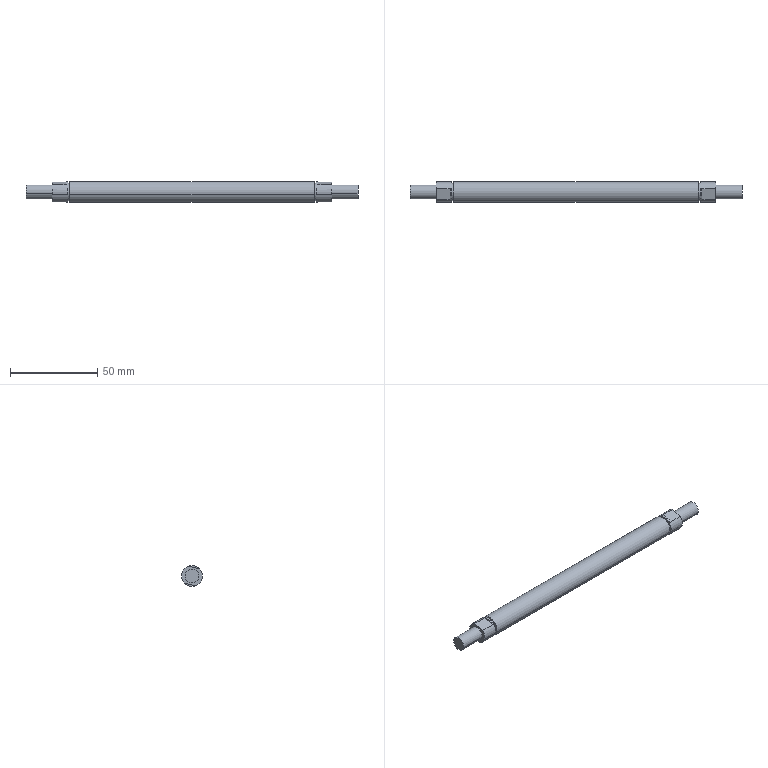Component | SolidWorks | IdlerAssembly4-1_RollerAxis3-1 | 1 solid | 30 faces | box 190 x 12 x 12 mm | volume 19390 mm3 | plane 16 | cylinder 14 | commonest cylinder face diameters 12 x6 10 x4 8 x4
build123d program:
from build123d import *

# Parameters (mm, degrees)
SKETCH1_R           = 6
BOSS_EXTRUDE1_DEPTH = 80
SKETCH3_R           = 4
BOSS_EXTRUDE2_DEPTH = 15
CUT_EXTRUDE7_START  = -8
CUT_EXTRUDE7_DEPTH  = 8
SKETCH20_W          = 1
SKETCH20_H          = 1


with BuildPart() as part:
    # Sketch1 → Boss-Extrude1 (new body)
    with BuildSketch(Plane(origin=(0, 0, 0), x_dir=(1, 0, 0), z_dir=(0, 1, 0))):
        with Locations(Location((0, 0, 0), (0, 0, 270))):
            Circle(SKETCH1_R)
    extrude(amount=BOSS_EXTRUDE1_DEPTH)

    # Sketch3 → Boss-Extrude2 (add)
    with BuildSketch(Plane(origin=(0, 80, 0), x_dir=(1, 0, 0), z_dir=(0, 1, 0))):
        with Locations(Location((0, 0, 0), (0, 0, 270))):
            Circle(SKETCH3_R)
    extrude(amount=BOSS_EXTRUDE2_DEPTH)

    # Sketch17 → Cut-Extrude7 (cut)
    with BuildSketch(Plane(origin=(0, 80, 0), x_dir=(1, 0, 0), z_dir=(0, 1, 0)).offset(CUT_EXTRUDE7_START)):
        with BuildLine():
            Line((-5, 3.317), (-5, -3.317))
            ThreePointArc((-5, -3.317), (-6, 0), (-5, 3.317))
        make_face()
        with BuildLine():
            Line((5, 3.317), (5, -3.317))
            ThreePointArc((5, -3.317), (6, 0), (5, 3.317))
        make_face()
    extrude(amount=CUT_EXTRUDE7_DEPTH, mode=Mode.SUBTRACT)

    # Sketch20 → Cut-Revolve1 (revolve, cut)
    with BuildSketch(Plane(origin=(0, 0, 0), x_dir=(0, 0, -1), z_dir=(1, 0, 0)), mode=Mode.PRIVATE) as cut_revolve1_sk:
        with Locations((5.5, 70.5)):
            Rectangle(SKETCH20_W, SKETCH20_H)
    revolve(cut_revolve1_sk.sketch.rotate(Axis((0, 95, 0), (0, -1, 0)), 180), axis=Axis((0, 95, 0), (0, -1, 0)), mode=Mode.SUBTRACT)

    # Mirror1: part across plane


with BuildPart() as part_1:
    add(part.part)
    add(part.part.mirror(Plane.ZX))


solid = part_1.part

# Placed as in the assembly
solid = solid.moved(Location((-244.97, -95, 30), (-75.719, 0, -90)))
STEP:
#1=COLOUR_RGB('',0.7922,0.8196,0.9333);
#2=FILL_AREA_STYLE_COLOUR('',#1);
#3=FILL_AREA_STYLE('',(#2));
#4=SURFACE_STYLE_FILL_AREA(#3);
#5=SURFACE_SIDE_STYLE('',(#4));
#6=SURFACE_STYLE_USAGE(.BOTH.,#5);
#7=PRESENTATION_STYLE_ASSIGNMENT((#6));
#8=CARTESIAN_POINT('',(-12.4,-3.931,1.133));
#9=VERTEX_POINT('',#8);
#10=CARTESIAN_POINT('',(-12.4,-3.549,1.23));
#11=VERTEX_POINT('',#10);
#12=CARTESIAN_POINT('',(-12.4,-3.74,1.181));
#13=DIRECTION('',(1.,0.,0.));
#14=DIRECTION('',(0.,0.9691,0.2467));
#15=AXIS2_PLACEMENT_3D('',#12,#13,#14);
#16=CIRCLE('',#15,0.1969);
#17=EDGE_CURVE('',#9,#11,#16,.T.);
#18=ORIENTED_EDGE('',*,*,#17,.F.);
#19=CARTESIAN_POINT('',(-12.44,-3.931,1.133));
#20=VERTEX_POINT('',#19);
#21=CARTESIAN_POINT('',(-13.385,-3.931,1.133));
#22=DIRECTION('',(-1.,-0.,-0.));
#23=VECTOR('',#22,39.37);
#24=LINE('',#21,#23);
#25=EDGE_CURVE('',#9,#20,#24,.T.);
#26=ORIENTED_EDGE('',*,*,#25,.T.);
#27=CARTESIAN_POINT('',(-12.44,-3.549,1.23));
#28=VERTEX_POINT('',#27);
#29=CARTESIAN_POINT('',(-12.44,-3.74,1.181));
#30=DIRECTION('',(1.,0.,0.));
#31=DIRECTION('',(0.,0.9691,0.2467));
#32=AXIS2_PLACEMENT_3D('',#29,#30,#31);
#33=CIRCLE('',#32,0.1969);
#34=EDGE_CURVE('',#20,#28,#33,.T.);
#35=ORIENTED_EDGE('',*,*,#34,.T.);
#36=CARTESIAN_POINT('',(-13.385,-3.549,1.23));
#37=DIRECTION('',(-1.,-0.,-0.));
#38=VECTOR('',#37,39.37);
#39=LINE('',#36,#38);
#40=EDGE_CURVE('',#11,#28,#39,.T.);
#41=ORIENTED_EDGE('',*,*,#40,.F.);
#42=EDGE_LOOP('',(#18,#26,#35,#41));
#43=FACE_OUTER_BOUND('',#42,.T.);
#44=CARTESIAN_POINT('',(-13.385,-3.74,1.181));
#45=DIRECTION('',(-1.,-0.,-0.));
#46=DIRECTION('',(0.,0.9691,0.2467));
#47=AXIS2_PLACEMENT_3D('',#44,#45,#46);
#48=CYLINDRICAL_SURFACE('',#47,0.1969);
#49=ADVANCED_FACE('',(#43),#48,.T.);
#50=CARTESIAN_POINT('',(-13.385,-3.893,1.142));
#51=VERTEX_POINT('',#50);
#52=CARTESIAN_POINT('',(-13.385,-3.588,1.22));
#53=VERTEX_POINT('',#52);
#54=CARTESIAN_POINT('',(-13.385,-3.74,1.181));
#55=DIRECTION('',(1.,0.,0.));
#56=DIRECTION('',(0.,0.9691,0.2467));
#57=AXIS2_PLACEMENT_3D('',#54,#55,#56);
#58=CIRCLE('',#57,0.1575);
#59=EDGE_CURVE('',#51,#53,#58,.T.);
#60=ORIENTED_EDGE('',*,*,#59,.T.);
#61=CARTESIAN_POINT('',(-12.794,-3.588,1.22));
#62=VERTEX_POINT('',#61);
#63=CARTESIAN_POINT('',(-13.385,-3.588,1.22));
#64=DIRECTION('',(1.,0.,0.));
#65=VECTOR('',#64,39.37);
#66=LINE('',#63,#65);
#67=EDGE_CURVE('',#53,#62,#66,.T.);
#68=ORIENTED_EDGE('',*,*,#67,.T.);
#69=CARTESIAN_POINT('',(-12.794,-3.893,1.142));
#70=VERTEX_POINT('',#69);
#71=CARTESIAN_POINT('',(-12.794,-3.74,1.181));
#72=DIRECTION('',(1.,0.,0.));
#73=DIRECTION('',(0.,0.9691,0.2467));
#74=AXIS2_PLACEMENT_3D('',#71,#72,#73);
#75=CIRCLE('',#74,0.1575);
#76=EDGE_CURVE('',#70,#62,#75,.T.);
#77=ORIENTED_EDGE('',*,*,#76,.F.);
#78=CARTESIAN_POINT('',(-13.385,-3.893,1.142));
#79=DIRECTION('',(1.,0.,0.));
#80=VECTOR('',#79,39.37);
#81=LINE('',#78,#80);
#82=EDGE_CURVE('',#51,#70,#81,.T.);
#83=ORIENTED_EDGE('',*,*,#82,.F.);
#84=EDGE_LOOP('',(#60,#68,#77,#83));
#85=FACE_OUTER_BOUND('',#84,.T.);
#86=CARTESIAN_POINT('',(-13.385,-3.74,1.181));
#87=DIRECTION('',(1.,0.,0.));
#88=DIRECTION('',(0.,-0.9691,-0.2467));
#89=AXIS2_PLACEMENT_3D('',#86,#87,#88);
#90=CYLINDRICAL_SURFACE('',#89,0.1575);
#91=ADVANCED_FACE('',(#85),#90,.T.);
#92=CARTESIAN_POINT('',(-12.794,-3.565,1.023));
#93=VERTEX_POINT('',#92);
#94=CARTESIAN_POINT('',(-12.794,-3.511,1.239));
#95=VERTEX_POINT('',#94);
#96=CARTESIAN_POINT('',(-12.794,-3.74,1.181));
#97=DIRECTION('',(1.,0.,0.));
#98=DIRECTION('',(0.,0.9691,0.2467));
#99=AXIS2_PLACEMENT_3D('',#96,#97,#98);
#100=CIRCLE('',#99,0.2362);
#101=EDGE_CURVE('',#93,#95,#100,.T.);
#102=ORIENTED_EDGE('',*,*,#101,.T.);
#103=CARTESIAN_POINT('',(-12.44,-3.511,1.239));
#104=VERTEX_POINT('',#103);
#105=CARTESIAN_POINT('',(-12.794,-3.511,1.239));
#106=DIRECTION('',(1.,0.,0.));
#107=VECTOR('',#106,39.37);
#108=LINE('',#105,#107);
#109=EDGE_CURVE('',#95,#104,#108,.T.);
#110=ORIENTED_EDGE('',*,*,#109,.T.);
#111=CARTESIAN_POINT('',(-12.44,-3.969,1.123));
#112=VERTEX_POINT('',#111);
#113=CARTESIAN_POINT('',(-12.44,-3.74,1.181));
#114=DIRECTION('',(1.,0.,0.));
#115=DIRECTION('',(0.,0.9691,0.2467));
#116=AXIS2_PLACEMENT_3D('',#113,#114,#115);
#117=CIRCLE('',#116,0.2362);
#118=EDGE_CURVE('',#112,#104,#117,.T.);
#119=ORIENTED_EDGE('',*,*,#118,.F.);
#120=CARTESIAN_POINT('',(-12.794,-3.969,1.123));
#121=VERTEX_POINT('',#120);
#122=CARTESIAN_POINT('',(-12.794,-3.969,1.123));
#123=DIRECTION('',(1.,0.,0.));
#124=VECTOR('',#123,39.37);
#125=LINE('',#122,#124);
#126=EDGE_CURVE('',#121,#112,#125,.T.);
#127=ORIENTED_EDGE('',*,*,#126,.F.);
#128=CARTESIAN_POINT('',(-12.794,-3.818,0.9581));
#129=VERTEX_POINT('',#128);
#130=CARTESIAN_POINT('',(-12.794,-3.74,1.181));
#131=DIRECTION('',(1.,0.,0.));
#132=DIRECTION('',(0.,0.9691,0.2467));
#133=AXIS2_PLACEMENT_3D('',#130,#131,#132);
#134=CIRCLE('',#133,0.2362);
#135=EDGE_CURVE('',#121,#129,#134,.T.);
#136=ORIENTED_EDGE('',*,*,#135,.T.);
#137=CARTESIAN_POINT('',(-12.479,-3.818,0.9581));
#138=VERTEX_POINT('',#137);
#139=CARTESIAN_POINT('',(-12.479,-3.818,0.9581));
#140=DIRECTION('',(-1.,-0.,-0.));
#141=VECTOR('',#140,39.37);
#142=LINE('',#139,#141);
#143=EDGE_CURVE('',#138,#129,#142,.T.);
#144=ORIENTED_EDGE('',*,*,#143,.F.);
#145=CARTESIAN_POINT('',(-12.479,-3.565,1.023));
#146=VERTEX_POINT('',#145);
#147=CARTESIAN_POINT('',(-12.479,-3.74,1.181));
#148=DIRECTION('',(1.,0.,0.));
#149=DIRECTION('',(0.,0.9691,0.2467));
#150=AXIS2_PLACEMENT_3D('',#147,#148,#149);
#151=CIRCLE('',#150,0.2362);
#152=EDGE_CURVE('',#138,#146,#151,.T.);
#153=ORIENTED_EDGE('',*,*,#152,.T.);
#154=CARTESIAN_POINT('',(-12.479,-3.565,1.023));
#155=DIRECTION('',(-1.,-0.,-0.));
#156=VECTOR('',#155,39.37);
#157=LINE('',#154,#156);
#158=EDGE_CURVE('',#146,#93,#157,.T.);
#159=ORIENTED_EDGE('',*,*,#158,.T.);
#160=EDGE_LOOP('',(#102,#110,#119,#127,#136,#144,#153,#159));
#161=FACE_OUTER_BOUND('',#160,.T.);
#162=CARTESIAN_POINT('',(-12.794,-3.74,1.181));
#163=DIRECTION('',(1.,0.,0.));
#164=DIRECTION('',(0.,-0.9691,-0.2467));
#165=AXIS2_PLACEMENT_3D('',#162,#163,#164);
#166=CYLINDRICAL_SURFACE('',#165,0.2362);
#167=ADVANCED_FACE('',(#161),#166,.T.);
#168=CARTESIAN_POINT('',(-6.889,-3.511,1.239));
#169=VERTEX_POINT('',#168);
#170=CARTESIAN_POINT('',(-6.889,-3.969,1.123));
#171=VERTEX_POINT('',#170);
#172=CARTESIAN_POINT('',(-6.889,-3.74,1.181));
#173=DIRECTION('',(1.,0.,0.));
#174=DIRECTION('',(0.,0.9691,0.2467));
#175=AXIS2_PLACEMENT_3D('',#172,#173,#174);
#176=CIRCLE('',#175,0.2362);
#177=EDGE_CURVE('',#169,#171,#176,.T.);
#178=ORIENTED_EDGE('',*,*,#177,.F.);
#179=CARTESIAN_POINT('',(-12.4,-3.511,1.239));
#180=VERTEX_POINT('',#179);
#181=CARTESIAN_POINT('',(-6.495,-3.511,1.239));
#182=DIRECTION('',(-1.,-0.,-0.));
#183=VECTOR('',#182,39.37);
#184=LINE('',#181,#183);
#185=EDGE_CURVE('',#169,#180,#184,.T.);
#186=ORIENTED_EDGE('',*,*,#185,.T.);
#187=CARTESIAN_POINT('',(-12.4,-3.969,1.123));
#188=VERTEX_POINT('',#187);
#189=CARTESIAN_POINT('',(-12.4,-3.74,1.181));
#190=DIRECTION('',(1.,0.,0.));
#191=DIRECTION('',(0.,0.9691,0.2467));
#192=AXIS2_PLACEMENT_3D('',#189,#190,#191);
#193=CIRCLE('',#192,0.2362);
#194=EDGE_CURVE('',#180,#188,#193,.T.);
#195=ORIENTED_EDGE('',*,*,#194,.T.);
#196=CARTESIAN_POINT('',(-6.495,-3.969,1.123));
#197=DIRECTION('',(-1.,-0.,-0.));
#198=VECTOR('',#197,39.37);
#199=LINE('',#196,#198);
#200=EDGE_CURVE('',#171,#188,#199,.T.);
#201=ORIENTED_EDGE('',*,*,#200,.F.);
#202=EDGE_LOOP('',(#178,#186,#195,#201));
#203=FACE_OUTER_BOUND('',#202,.T.);
#204=CARTESIAN_POINT('',(-6.495,-3.74,1.181));
#205=DIRECTION('',(-1.,-0.,-0.));
#206=DIRECTION('',(0.,-0.9691,-0.2467));
#207=AXIS2_PLACEMENT_3D('',#204,#205,#206);
#208=CYLINDRICAL_SURFACE('',#207,0.2362);
#209=ADVANCED_FACE('',(#203),#208,.T.);
#210=CARTESIAN_POINT('',(-6.889,-3.549,1.23));
#211=VERTEX_POINT('',#210);
#212=CARTESIAN_POINT('',(-6.889,-3.931,1.133));
#213=VERTEX_POINT('',#212);
#214=CARTESIAN_POINT('',(-6.889,-3.74,1.181));
#215=DIRECTION('',(1.,0.,0.));
#216=DIRECTION('',(0.,0.9691,0.2467));
#217=AXIS2_PLACEMENT_3D('',#214,#215,#216);
#218=CIRCLE('',#217,0.1969);
#219=EDGE_CURVE('',#211,#213,#218,.T.);
#220=ORIENTED_EDGE('',*,*,#219,.T.);
#221=CARTESIAN_POINT('',(-6.849,-3.931,1.133));
#222=VERTEX_POINT('',#221);
#223=CARTESIAN_POINT('',(-5.904,-3.931,1.133));
#224=DIRECTION('',(1.,0.,0.));
#225=VECTOR('',#224,39.37);
#226=LINE('',#223,#225);
#227=EDGE_CURVE('',#213,#222,#226,.T.);
#228=ORIENTED_EDGE('',*,*,#227,.T.);
#229=CARTESIAN_POINT('',(-6.849,-3.549,1.23));
#230=VERTEX_POINT('',#229);
#231=CARTESIAN_POINT('',(-6.849,-3.74,1.181));
#232=DIRECTION('',(1.,0.,0.));
#233=DIRECTION('',(0.,0.9691,0.2467));
#234=AXIS2_PLACEMENT_3D('',#231,#232,#233);
#235=CIRCLE('',#234,0.1969);
#236=EDGE_CURVE('',#230,#222,#235,.T.);
#237=ORIENTED_EDGE('',*,*,#236,.F.);
#238=CARTESIAN_POINT('',(-5.904,-3.549,1.23));
#239=DIRECTION('',(1.,0.,0.));
#240=VECTOR('',#239,39.37);
#241=LINE('',#238,#240);
#242=EDGE_CURVE('',#211,#230,#241,.T.);
#243=ORIENTED_EDGE('',*,*,#242,.F.);
#244=EDGE_LOOP('',(#220,#228,#237,#243));
#245=FACE_OUTER_BOUND('',#244,.T.);
#246=CARTESIAN_POINT('',(-5.904,-3.74,1.181));
#247=DIRECTION('',(1.,0.,0.));
#248=DIRECTION('',(0.,0.9691,0.2467));
#249=AXIS2_PLACEMENT_3D('',#246,#247,#248);
#250=CYLINDRICAL_SURFACE('',#249,0.1969);
#251=ADVANCED_FACE('',(#245),#250,.T.);
#252=CARTESIAN_POINT('',(-5.904,-3.588,1.22));
#253=VERTEX_POINT('',#252);
#254=CARTESIAN_POINT('',(-5.904,-3.893,1.142));
#255=VERTEX_POINT('',#254);
#256=CARTESIAN_POINT('',(-5.904,-3.74,1.181));
#257=DIRECTION('',(1.,0.,0.));
#258=DIRECTION('',(0.,0.9691,0.2467));
#259=AXIS2_PLACEMENT_3D('',#256,#257,#258);
#260=CIRCLE('',#259,0.1575);
#261=EDGE_CURVE('',#253,#255,#260,.T.);
#262=ORIENTED_EDGE('',*,*,#261,.F.);
#263=CARTESIAN_POINT('',(-6.495,-3.588,1.22));
#264=VERTEX_POINT('',#263);
#265=CARTESIAN_POINT('',(-5.904,-3.588,1.22));
#266=DIRECTION('',(-1.,-0.,-0.));
#267=VECTOR('',#266,39.37);
#268=LINE('',#265,#267);
#269=EDGE_CURVE('',#253,#264,#268,.T.);
#270=ORIENTED_EDGE('',*,*,#269,.T.);
#271=CARTESIAN_POINT('',(-6.495,-3.893,1.142));
#272=VERTEX_POINT('',#271);
#273=CARTESIAN_POINT('',(-6.495,-3.74,1.181));
#274=DIRECTION('',(1.,0.,0.));
#275=DIRECTION('',(0.,0.9691,0.2467));
#276=AXIS2_PLACEMENT_3D('',#273,#274,#275);
#277=CIRCLE('',#276,0.1575);
#278=EDGE_CURVE('',#264,#272,#277,.T.);
#279=ORIENTED_EDGE('',*,*,#278,.T.);
#280=CARTESIAN_POINT('',(-5.904,-3.893,1.142));
#281=DIRECTION('',(-1.,-0.,-0.));
#282=VECTOR('',#281,39.37);
#283=LINE('',#280,#282);
#284=EDGE_CURVE('',#255,#272,#283,.T.);
#285=ORIENTED_EDGE('',*,*,#284,.F.);
#286=EDGE_LOOP('',(#262,#270,#279,#285));
#287=FACE_OUTER_BOUND('',#286,.T.);
#288=CARTESIAN_POINT('',(-5.904,-3.74,1.181));
#289=DIRECTION('',(-1.,-0.,-0.));
#290=DIRECTION('',(0.,-0.9691,-0.2467));
#291=AXIS2_PLACEMENT_3D('',#288,#289,#290);
#292=CYLINDRICAL_SURFACE('',#291,0.1575);
#293=ADVANCED_FACE('',(#287),#292,.T.);
#294=CARTESIAN_POINT('',(-6.495,-3.511,1.239));
#295=VERTEX_POINT('',#294);
#296=CARTESIAN_POINT('',(-6.495,-3.662,1.404));
#297=VERTEX_POINT('',#296);
#298=CARTESIAN_POINT('',(-6.495,-3.74,1.181));
#299=DIRECTION('',(1.,0.,0.));
#300=DIRECTION('',(0.,0.9691,0.2467));
#301=AXIS2_PLACEMENT_3D('',#298,#299,#300);
#302=CIRCLE('',#301,0.2362);
#303=EDGE_CURVE('',#295,#297,#302,.T.);
#304=ORIENTED_EDGE('',*,*,#303,.F.);
#305=CARTESIAN_POINT('',(-6.849,-3.511,1.239));
#306=VERTEX_POINT('',#305);
#307=CARTESIAN_POINT('',(-6.495,-3.511,1.239));
#308=DIRECTION('',(-1.,-0.,-0.));
#309=VECTOR('',#308,39.37);
#310=LINE('',#307,#309);
#311=EDGE_CURVE('',#295,#306,#310,.T.);
#312=ORIENTED_EDGE('',*,*,#311,.T.);
#313=CARTESIAN_POINT('',(-6.849,-3.969,1.123));
#314=VERTEX_POINT('',#313);
#315=CARTESIAN_POINT('',(-6.849,-3.74,1.181));
#316=DIRECTION('',(1.,0.,0.));
#317=DIRECTION('',(0.,0.9691,0.2467));
#318=AXIS2_PLACEMENT_3D('',#315,#316,#317);
#319=CIRCLE('',#318,0.2362);
#320=EDGE_CURVE('',#306,#314,#319,.T.);
#321=ORIENTED_EDGE('',*,*,#320,.T.);
#322=CARTESIAN_POINT('',(-6.495,-3.969,1.123));
#323=VERTEX_POINT('',#322);
#324=CARTESIAN_POINT('',(-6.495,-3.969,1.123));
#325=DIRECTION('',(-1.,-0.,-0.));
#326=VECTOR('',#325,39.37);
#327=LINE('',#324,#326);
#328=EDGE_CURVE('',#323,#314,#327,.T.);
#329=ORIENTED_EDGE('',*,*,#328,.F.);
#330=CARTESIAN_POINT('',(-6.495,-3.915,1.34));
#331=VERTEX_POINT('',#330);
#332=CARTESIAN_POINT('',(-6.495,-3.74,1.181));
#333=DIRECTION('',(1.,0.,0.));
#334=DIRECTION('',(0.,0.9691,0.2467));
#335=AXIS2_PLACEMENT_3D('',#332,#333,#334);
#336=CIRCLE('',#335,0.2362);
#337=EDGE_CURVE('',#331,#323,#336,.T.);
#338=ORIENTED_EDGE('',*,*,#337,.F.);
#339=CARTESIAN_POINT('',(-6.81,-3.915,1.34));
#340=VERTEX_POINT('',#339);
#341=CARTESIAN_POINT('',(-6.81,-3.915,1.34));
#342=DIRECTION('',(1.,0.,0.));
#343=VECTOR('',#342,39.37);
#344=LINE('',#341,#343);
#345=EDGE_CURVE('',#340,#331,#344,.T.);
#346=ORIENTED_EDGE('',*,*,#345,.F.);
#347=CARTESIAN_POINT('',(-6.81,-3.662,1.404));
#348=VERTEX_POINT('',#347);
#349=CARTESIAN_POINT('',(-6.81,-3.74,1.181));
#350=DIRECTION('',(1.,0.,0.));
#351=DIRECTION('',(0.,0.9691,0.2467));
#352=AXIS2_PLACEMENT_3D('',#349,#350,#351);
#353=CIRCLE('',#352,0.2362);
#354=EDGE_CURVE('',#348,#340,#353,.T.);
#355=ORIENTED_EDGE('',*,*,#354,.F.);
#356=CARTESIAN_POINT('',(-6.81,-3.662,1.404));
#357=DIRECTION('',(1.,0.,0.));
#358=VECTOR('',#357,39.37);
#359=LINE('',#356,#358);
#360=EDGE_CURVE('',#348,#297,#359,.T.);
#361=ORIENTED_EDGE('',*,*,#360,.T.);
#362=EDGE_LOOP('',(#304,#312,#321,#329,#338,#346,#355,#361));
#363=FACE_OUTER_BOUND('',#362,.T.);
#364=CARTESIAN_POINT('',(-6.495,-3.74,1.181));
#365=DIRECTION('',(-1.,-0.,-0.));
#366=DIRECTION('',(0.,-0.9691,-0.2467));
#367=AXIS2_PLACEMENT_3D('',#364,#365,#366);
#368=CYLINDRICAL_SURFACE('',#367,0.2362);
#369=ADVANCED_FACE('',(#363),#368,.T.);
#370=ORIENTED_EDGE('',*,*,#311,.F.);
#371=CARTESIAN_POINT('',(-6.495,-3.565,1.023));
#372=VERTEX_POINT('',#371);
#373=CARTESIAN_POINT('',(-6.495,-3.74,1.181));
#374=DIRECTION('',(1.,0.,0.));
#375=DIRECTION('',(0.,0.9691,0.2467));
#376=AXIS2_PLACEMENT_3D('',#373,#374,#375);
#377=CIRCLE('',#376,0.2362);
#378=EDGE_CURVE('',#372,#295,#377,.T.);
#379=ORIENTED_EDGE('',*,*,#378,.F.);
#380=CARTESIAN_POINT('',(-6.81,-3.565,1.023));
#381=VERTEX_POINT('',#380);
#382=CARTESIAN_POINT('',(-6.81,-3.565,1.023));
#383=DIRECTION('',(1.,0.,0.));
#384=VECTOR('',#383,39.37);
#385=LINE('',#382,#384);
#386=EDGE_CURVE('',#381,#372,#385,.T.);
#387=ORIENTED_EDGE('',*,*,#386,.F.);
#388=CARTESIAN_POINT('',(-6.81,-3.818,0.9581));
#389=VERTEX_POINT('',#388);
#390=CARTESIAN_POINT('',(-6.81,-3.74,1.181));
#391=DIRECTION('',(1.,0.,0.));
#392=DIRECTION('',(0.,0.9691,0.2467));
#393=AXIS2_PLACEMENT_3D('',#390,#391,#392);
#394=CIRCLE('',#393,0.2362);
#395=EDGE_CURVE('',#389,#381,#394,.T.);
#396=ORIENTED_EDGE('',*,*,#395,.F.);
#397=CARTESIAN_POINT('',(-6.495,-3.818,0.9581));
#398=VERTEX_POINT('',#397);
#399=CARTESIAN_POINT('',(-6.81,-3.818,0.9581));
#400=DIRECTION('',(1.,0.,0.));
#401=VECTOR('',#400,39.37);
#402=LINE('',#399,#401);
#403=EDGE_CURVE('',#389,#398,#402,.T.);
#404=ORIENTED_EDGE('',*,*,#403,.T.);
#405=CARTESIAN_POINT('',(-6.495,-3.74,1.181));
#406=DIRECTION('',(1.,0.,0.));
#407=DIRECTION('',(0.,0.9691,0.2467));
#408=AXIS2_PLACEMENT_3D('',#405,#406,#407);
#409=CIRCLE('',#408,0.2362);
#410=EDGE_CURVE('',#323,#398,#409,.T.);
#411=ORIENTED_EDGE('',*,*,#410,.F.);
#412=ORIENTED_EDGE('',*,*,#328,.T.);
#413=CARTESIAN_POINT('',(-6.849,-3.74,1.181));
#414=DIRECTION('',(1.,0.,0.));
#415=DIRECTION('',(0.,0.9691,0.2467));
#416=AXIS2_PLACEMENT_3D('',#413,#414,#415);
#417=CIRCLE('',#416,0.2362);
#418=EDGE_CURVE('',#314,#306,#417,.T.);
#419=ORIENTED_EDGE('',*,*,#418,.T.);
#420=EDGE_LOOP('',(#370,#379,#387,#396,#404,#411,#412,#419));
#421=FACE_OUTER_BOUND('',#420,.T.);
#422=CARTESIAN_POINT('',(-6.495,-3.74,1.181));
#423=DIRECTION('',(-1.,-0.,-0.));
#424=DIRECTION('',(0.,-0.9691,-0.2467));
#425=AXIS2_PLACEMENT_3D('',#422,#423,#424);
#426=CYLINDRICAL_SURFACE('',#425,0.2362);
#427=ADVANCED_FACE('',(#421),#426,.T.);
#428=CARTESIAN_POINT('',(-6.495,-3.818,0.9581));
#429=DIRECTION('',(0.,-0.9691,-0.2467));
#430=VECTOR('',#429,39.37);
#431=LINE('',#428,#430);
#432=EDGE_CURVE('',#372,#398,#431,.T.);
#433=ORIENTED_EDGE('',*,*,#432,.F.);
#434=ORIENTED_EDGE('',*,*,#378,.T.);
#435=ORIENTED_EDGE('',*,*,#303,.T.);
#436=CARTESIAN_POINT('',(-6.495,-3.915,1.34));
#437=DIRECTION('',(-0.,0.9691,0.2467));
#438=VECTOR('',#437,39.37);
#439=LINE('',#436,#438);
#440=EDGE_CURVE('',#331,#297,#439,.T.);
#441=ORIENTED_EDGE('',*,*,#440,.F.);
#442=ORIENTED_EDGE('',*,*,#337,.T.);
#443=ORIENTED_EDGE('',*,*,#410,.T.);
#444=EDGE_LOOP('',(#433,#434,#435,#441,#442,#443));
#445=FACE_OUTER_BOUND('',#444,.T.);
#446=CARTESIAN_POINT('',(-6.495,-3.74,1.181));
#447=DIRECTION('',(1.,0.,0.));
#448=DIRECTION('',(0.,0.9691,0.2467));
#449=AXIS2_PLACEMENT_3D('',#446,#447,#448);
#450=CIRCLE('',#449,0.1575);
#451=EDGE_CURVE('',#272,#264,#450,.T.);
#452=ORIENTED_EDGE('',*,*,#451,.F.);
#453=ORIENTED_EDGE('',*,*,#278,.F.);
#454=EDGE_LOOP('',(#452,#453));
#455=FACE_BOUND('',#454,.T.);
#456=CARTESIAN_POINT('',(-6.495,-3.74,1.181));
#457=DIRECTION('',(1.,0.,0.));
#458=DIRECTION('',(-0.,0.9691,0.2467));
#459=AXIS2_PLACEMENT_3D('',#456,#457,#458);
#460=PLANE('',#459);
#461=ADVANCED_FACE('',(#445,#455),#460,.T.);
#462=ORIENTED_EDGE('',*,*,#269,.F.);
#463=CARTESIAN_POINT('',(-5.904,-3.74,1.181));
#464=DIRECTION('',(1.,0.,0.));
#465=DIRECTION('',(0.,0.9691,0.2467));
#466=AXIS2_PLACEMENT_3D('',#463,#464,#465);
#467=CIRCLE('',#466,0.1575);
#468=EDGE_CURVE('',#255,#253,#467,.T.);
#469=ORIENTED_EDGE('',*,*,#468,.F.);
#470=ORIENTED_EDGE('',*,*,#284,.T.);
#471=ORIENTED_EDGE('',*,*,#451,.T.);
#472=EDGE_LOOP('',(#462,#469,#470,#471));
#473=FACE_OUTER_BOUND('',#472,.T.);
#474=CARTESIAN_POINT('',(-5.904,-3.74,1.181));
#475=DIRECTION('',(-1.,-0.,-0.));
#476=DIRECTION('',(0.,-0.9691,-0.2467));
#477=AXIS2_PLACEMENT_3D('',#474,#475,#476);
#478=CYLINDRICAL_SURFACE('',#477,0.1575);
#479=ADVANCED_FACE('',(#473),#478,.T.);
#480=ORIENTED_EDGE('',*,*,#468,.T.);
#481=ORIENTED_EDGE('',*,*,#261,.T.);
#482=EDGE_LOOP('',(#480,#481));
#483=FACE_OUTER_BOUND('',#482,.T.);
#484=CARTESIAN_POINT('',(-5.904,-3.74,1.181));
#485=DIRECTION('',(1.,0.,0.));
#486=DIRECTION('',(-0.,0.9691,0.2467));
#487=AXIS2_PLACEMENT_3D('',#484,#485,#486);
#488=PLANE('',#487);
#489=ADVANCED_FACE('',(#483),#488,.T.);
#490=ORIENTED_EDGE('',*,*,#440,.T.);
#491=ORIENTED_EDGE('',*,*,#360,.F.);
#492=CARTESIAN_POINT('',(-6.81,-3.915,1.34));
#493=DIRECTION('',(-0.,0.9691,0.2467));
#494=VECTOR('',#493,39.37);
#495=LINE('',#492,#494);
#496=EDGE_CURVE('',#340,#348,#495,.T.);
#497=ORIENTED_EDGE('',*,*,#496,.F.);
#498=ORIENTED_EDGE('',*,*,#345,.T.);
#499=EDGE_LOOP('',(#490,#491,#497,#498));
#500=FACE_OUTER_BOUND('',#499,.T.);
#501=CARTESIAN_POINT('',(-6.81,-3.915,1.34));
#502=DIRECTION('',(0.,0.2467,-0.9691));
#503=DIRECTION('',(-0.,0.9691,0.2467));
#504=AXIS2_PLACEMENT_3D('',#501,#502,#503);
#505=PLANE('',#504);
#506=ADVANCED_FACE('',(#500),#505,.F.);
#507=ORIENTED_EDGE('',*,*,#354,.T.);
#508=ORIENTED_EDGE('',*,*,#496,.T.);
#509=EDGE_LOOP('',(#507,#508));
#510=FACE_OUTER_BOUND('',#509,.T.);
#511=CARTESIAN_POINT('',(-6.81,-3.74,1.181));
#512=DIRECTION('',(1.,0.,0.));
#513=DIRECTION('',(-0.,0.9691,0.2467));
#514=AXIS2_PLACEMENT_3D('',#511,#512,#513);
#515=PLANE('',#514);
#516=ADVANCED_FACE('',(#510),#515,.T.);
#517=ORIENTED_EDGE('',*,*,#432,.T.);
#518=ORIENTED_EDGE('',*,*,#403,.F.);
#519=CARTESIAN_POINT('',(-6.81,-3.818,0.9581));
#520=DIRECTION('',(0.,-0.9691,-0.2467));
#521=VECTOR('',#520,39.37);
#522=LINE('',#519,#521);
#523=EDGE_CURVE('',#381,#389,#522,.T.);
#524=ORIENTED_EDGE('',*,*,#523,.F.);
#525=ORIENTED_EDGE('',*,*,#386,.T.);
#526=EDGE_LOOP('',(#517,#518,#524,#525));
#527=FACE_OUTER_BOUND('',#526,.T.);
#528=CARTESIAN_POINT('',(-6.81,-3.818,0.9581));
#529=DIRECTION('',(-0.,-0.2467,0.9691));
#530=DIRECTION('',(0.,-0.9691,-0.2467));
#531=AXIS2_PLACEMENT_3D('',#528,#529,#530);
#532=PLANE('',#531);
#533=ADVANCED_FACE('',(#527),#532,.F.);
#534=ORIENTED_EDGE('',*,*,#395,.T.);
#535=ORIENTED_EDGE('',*,*,#523,.T.);
#536=EDGE_LOOP('',(#534,#535));
#537=FACE_OUTER_BOUND('',#536,.T.);
#538=CARTESIAN_POINT('',(-6.81,-3.74,1.181));
#539=DIRECTION('',(1.,0.,0.));
#540=DIRECTION('',(-0.,0.9691,0.2467));
#541=AXIS2_PLACEMENT_3D('',#538,#539,#540);
#542=PLANE('',#541);
#543=ADVANCED_FACE('',(#537),#542,.T.);
#544=CARTESIAN_POINT('',(-6.889,-3.74,1.181));
#545=DIRECTION('',(1.,0.,0.));
#546=DIRECTION('',(0.,0.9691,0.2467));
#547=AXIS2_PLACEMENT_3D('',#544,#545,#546);
#548=CIRCLE('',#547,0.2362);
#549=EDGE_CURVE('',#171,#169,#548,.T.);
#550=ORIENTED_EDGE('',*,*,#549,.T.);
#551=ORIENTED_EDGE('',*,*,#177,.T.);
#552=EDGE_LOOP('',(#550,#551));
#553=FACE_OUTER_BOUND('',#552,.T.);
#554=ORIENTED_EDGE('',*,*,#219,.F.);
#555=CARTESIAN_POINT('',(-6.889,-3.74,1.181));
#556=DIRECTION('',(1.,0.,0.));
#557=DIRECTION('',(0.,0.9691,0.2467));
#558=AXIS2_PLACEMENT_3D('',#555,#556,#557);
#559=CIRCLE('',#558,0.1969);
#560=EDGE_CURVE('',#213,#211,#559,.T.);
#561=ORIENTED_EDGE('',*,*,#560,.F.);
#562=EDGE_LOOP('',(#554,#561));
#563=FACE_BOUND('',#562,.T.);
#564=CARTESIAN_POINT('',(-6.889,-3.969,1.123));
#565=DIRECTION('',(1.,0.,0.));
#566=DIRECTION('',(-0.,0.9691,0.2467));
#567=AXIS2_PLACEMENT_3D('',#564,#565,#566);
#568=PLANE('',#567);
#569=ADVANCED_FACE('',(#553,#563),#568,.T.);
#570=ORIENTED_EDGE('',*,*,#227,.F.);
#571=ORIENTED_EDGE('',*,*,#560,.T.);
#572=ORIENTED_EDGE('',*,*,#242,.T.);
#573=CARTESIAN_POINT('',(-6.849,-3.74,1.181));
#574=DIRECTION('',(1.,0.,0.));
#575=DIRECTION('',(0.,0.9691,0.2467));
#576=AXIS2_PLACEMENT_3D('',#573,#574,#575);
#577=CIRCLE('',#576,0.1969);
#578=EDGE_CURVE('',#222,#230,#577,.T.);
#579=ORIENTED_EDGE('',*,*,#578,.F.);
#580=EDGE_LOOP('',(#570,#571,#572,#579));
#581=FACE_OUTER_BOUND('',#580,.T.);
#582=CARTESIAN_POINT('',(-5.904,-3.74,1.181));
#583=DIRECTION('',(1.,0.,0.));
#584=DIRECTION('',(0.,0.9691,0.2467));
#585=AXIS2_PLACEMENT_3D('',#582,#583,#584);
#586=CYLINDRICAL_SURFACE('',#585,0.1969);
#587=ADVANCED_FACE('',(#581),#586,.T.);
#588=ORIENTED_EDGE('',*,*,#236,.T.);
#589=ORIENTED_EDGE('',*,*,#578,.T.);
#590=EDGE_LOOP('',(#588,#589));
#591=FACE_BOUND('',#590,.T.);
#592=ORIENTED_EDGE('',*,*,#418,.F.);
#593=ORIENTED_EDGE('',*,*,#320,.F.);
#594=EDGE_LOOP('',(#592,#593));
#595=FACE_OUTER_BOUND('',#594,.T.);
#596=CARTESIAN_POINT('',(-6.849,-3.969,1.123));
#597=DIRECTION('',(-1.,-0.,-0.));
#598=DIRECTION('',(0.,-0.9691,-0.2467));
#599=AXIS2_PLACEMENT_3D('',#596,#597,#598);
#600=PLANE('',#599);
#601=ADVANCED_FACE('',(#591,#595),#600,.T.);
#602=ORIENTED_EDGE('',*,*,#185,.F.);
#603=ORIENTED_EDGE('',*,*,#549,.F.);
#604=ORIENTED_EDGE('',*,*,#200,.T.);
#605=CARTESIAN_POINT('',(-12.4,-3.74,1.181));
#606=DIRECTION('',(1.,0.,0.));
#607=DIRECTION('',(0.,0.9691,0.2467));
#608=AXIS2_PLACEMENT_3D('',#605,#606,#607);
#609=CIRCLE('',#608,0.2362);
#610=EDGE_CURVE('',#188,#180,#609,.T.);
#611=ORIENTED_EDGE('',*,*,#610,.T.);
#612=EDGE_LOOP('',(#602,#603,#604,#611));
#613=FACE_OUTER_BOUND('',#612,.T.);
#614=CARTESIAN_POINT('',(-6.495,-3.74,1.181));
#615=DIRECTION('',(-1.,-0.,-0.));
#616=DIRECTION('',(0.,-0.9691,-0.2467));
#617=AXIS2_PLACEMENT_3D('',#614,#615,#616);
#618=CYLINDRICAL_SURFACE('',#617,0.2362);
#619=ADVANCED_FACE('',(#613),#618,.T.);
#620=ORIENTED_EDGE('',*,*,#109,.F.);
#621=CARTESIAN_POINT('',(-12.794,-3.662,1.404));
#622=VERTEX_POINT('',#621);
#623=CARTESIAN_POINT('',(-12.794,-3.74,1.181));
#624=DIRECTION('',(1.,0.,0.));
#625=DIRECTION('',(0.,0.9691,0.2467));
#626=AXIS2_PLACEMENT_3D('',#623,#624,#625);
#627=CIRCLE('',#626,0.2362);
#628=EDGE_CURVE('',#95,#622,#627,.T.);
#629=ORIENTED_EDGE('',*,*,#628,.T.);
#630=CARTESIAN_POINT('',(-12.479,-3.662,1.404));
#631=VERTEX_POINT('',#630);
#632=CARTESIAN_POINT('',(-12.479,-3.662,1.404));
#633=DIRECTION('',(-1.,-0.,-0.));
#634=VECTOR('',#633,39.37);
#635=LINE('',#632,#634);
#636=EDGE_CURVE('',#631,#622,#635,.T.);
#637=ORIENTED_EDGE('',*,*,#636,.F.);
#638=CARTESIAN_POINT('',(-12.479,-3.915,1.34));
#639=VERTEX_POINT('',#638);
#640=CARTESIAN_POINT('',(-12.479,-3.74,1.181));
#641=DIRECTION('',(1.,0.,0.));
#642=DIRECTION('',(0.,0.9691,0.2467));
#643=AXIS2_PLACEMENT_3D('',#640,#641,#642);
#644=CIRCLE('',#643,0.2362);
#645=EDGE_CURVE('',#631,#639,#644,.T.);
#646=ORIENTED_EDGE('',*,*,#645,.T.);
#647=CARTESIAN_POINT('',(-12.794,-3.915,1.34));
#648=VERTEX_POINT('',#647);
#649=CARTESIAN_POINT('',(-12.479,-3.915,1.34));
#650=DIRECTION('',(-1.,-0.,-0.));
#651=VECTOR('',#650,39.37);
#652=LINE('',#649,#651);
#653=EDGE_CURVE('',#639,#648,#652,.T.);
#654=ORIENTED_EDGE('',*,*,#653,.T.);
#655=CARTESIAN_POINT('',(-12.794,-3.74,1.181));
#656=DIRECTION('',(1.,0.,0.));
#657=DIRECTION('',(0.,0.9691,0.2467));
#658=AXIS2_PLACEMENT_3D('',#655,#656,#657);
#659=CIRCLE('',#658,0.2362);
#660=EDGE_CURVE('',#648,#121,#659,.T.);
#661=ORIENTED_EDGE('',*,*,#660,.T.);
#662=ORIENTED_EDGE('',*,*,#126,.T.);
#663=CARTESIAN_POINT('',(-12.44,-3.74,1.181));
#664=DIRECTION('',(1.,0.,0.));
#665=DIRECTION('',(0.,0.9691,0.2467));
#666=AXIS2_PLACEMENT_3D('',#663,#664,#665);
#667=CIRCLE('',#666,0.2362);
#668=EDGE_CURVE('',#104,#112,#667,.T.);
#669=ORIENTED_EDGE('',*,*,#668,.F.);
#670=EDGE_LOOP('',(#620,#629,#637,#646,#654,#661,#662,#669));
#671=FACE_OUTER_BOUND('',#670,.T.);
#672=CARTESIAN_POINT('',(-12.794,-3.74,1.181));
#673=DIRECTION('',(1.,0.,0.));
#674=DIRECTION('',(0.,-0.9691,-0.2467));
#675=AXIS2_PLACEMENT_3D('',#672,#673,#674);
#676=CYLINDRICAL_SURFACE('',#675,0.2362);
#677=ADVANCED_FACE('',(#671),#676,.T.);
#678=CARTESIAN_POINT('',(-12.794,-3.818,0.9581));
#679=DIRECTION('',(0.,-0.9691,-0.2467));
#680=VECTOR('',#679,39.37);
#681=LINE('',#678,#680);
#682=EDGE_CURVE('',#93,#129,#681,.T.);
#683=ORIENTED_EDGE('',*,*,#682,.T.);
#684=ORIENTED_EDGE('',*,*,#135,.F.);
#685=ORIENTED_EDGE('',*,*,#660,.F.);
#686=CARTESIAN_POINT('',(-12.794,-3.915,1.34));
#687=DIRECTION('',(-0.,0.9691,0.2467));
#688=VECTOR('',#687,39.37);
#689=LINE('',#686,#688);
#690=EDGE_CURVE('',#648,#622,#689,.T.);
#691=ORIENTED_EDGE('',*,*,#690,.T.);
#692=ORIENTED_EDGE('',*,*,#628,.F.);
#693=ORIENTED_EDGE('',*,*,#101,.F.);
#694=EDGE_LOOP('',(#683,#684,#685,#691,#692,#693));
#695=FACE_OUTER_BOUND('',#694,.T.);
#696=ORIENTED_EDGE('',*,*,#76,.T.);
#697=CARTESIAN_POINT('',(-12.794,-3.74,1.181));
#698=DIRECTION('',(1.,0.,0.));
#699=DIRECTION('',(0.,0.9691,0.2467));
#700=AXIS2_PLACEMENT_3D('',#697,#698,#699);
#701=CIRCLE('',#700,0.1575);
#702=EDGE_CURVE('',#62,#70,#701,.T.);
#703=ORIENTED_EDGE('',*,*,#702,.T.);
#704=EDGE_LOOP('',(#696,#703));
#705=FACE_BOUND('',#704,.T.);
#706=CARTESIAN_POINT('',(-12.794,-3.74,1.181));
#707=DIRECTION('',(-1.,-0.,-0.));
#708=DIRECTION('',(-0.,0.9691,0.2467));
#709=AXIS2_PLACEMENT_3D('',#706,#707,#708);
#710=PLANE('',#709);
#711=ADVANCED_FACE('',(#695,#705),#710,.T.);
#712=ORIENTED_EDGE('',*,*,#67,.F.);
#713=CARTESIAN_POINT('',(-13.385,-3.74,1.181));
#714=DIRECTION('',(1.,0.,0.));
#715=DIRECTION('',(0.,0.9691,0.2467));
#716=AXIS2_PLACEMENT_3D('',#713,#714,#715);
#717=CIRCLE('',#716,0.1575);
#718=EDGE_CURVE('',#53,#51,#717,.T.);
#719=ORIENTED_EDGE('',*,*,#718,.T.);
#720=ORIENTED_EDGE('',*,*,#82,.T.);
#721=ORIENTED_EDGE('',*,*,#702,.F.);
#722=EDGE_LOOP('',(#712,#719,#720,#721));
#723=FACE_OUTER_BOUND('',#722,.T.);
#724=CARTESIAN_POINT('',(-13.385,-3.74,1.181));
#725=DIRECTION('',(1.,0.,0.));
#726=DIRECTION('',(0.,-0.9691,-0.2467));
#727=AXIS2_PLACEMENT_3D('',#724,#725,#726);
#728=CYLINDRICAL_SURFACE('',#727,0.1575);
#729=ADVANCED_FACE('',(#723),#728,.T.);
#730=ORIENTED_EDGE('',*,*,#59,.F.);
#731=ORIENTED_EDGE('',*,*,#718,.F.);
#732=EDGE_LOOP('',(#730,#731));
#733=FACE_OUTER_BOUND('',#732,.T.);
#734=CARTESIAN_POINT('',(-13.385,-3.74,1.181));
#735=DIRECTION('',(-1.,-0.,-0.));
#736=DIRECTION('',(-0.,0.9691,0.2467));
#737=AXIS2_PLACEMENT_3D('',#734,#735,#736);
#738=PLANE('',#737);
#739=ADVANCED_FACE('',(#733),#738,.T.);
#740=ORIENTED_EDGE('',*,*,#690,.F.);
#741=ORIENTED_EDGE('',*,*,#653,.F.);
#742=CARTESIAN_POINT('',(-12.479,-3.915,1.34));
#743=DIRECTION('',(-0.,0.9691,0.2467));
#744=VECTOR('',#743,39.37);
#745=LINE('',#742,#744);
#746=EDGE_CURVE('',#639,#631,#745,.T.);
#747=ORIENTED_EDGE('',*,*,#746,.T.);
#748=ORIENTED_EDGE('',*,*,#636,.T.);
#749=EDGE_LOOP('',(#740,#741,#747,#748));
#750=FACE_OUTER_BOUND('',#749,.T.);
#751=CARTESIAN_POINT('',(-12.479,-3.915,1.34));
#752=DIRECTION('',(0.,0.2467,-0.9691));
#753=DIRECTION('',(-0.,0.9691,0.2467));
#754=AXIS2_PLACEMENT_3D('',#751,#752,#753);
#755=PLANE('',#754);
#756=ADVANCED_FACE('',(#750),#755,.F.);
#757=ORIENTED_EDGE('',*,*,#645,.F.);
#758=ORIENTED_EDGE('',*,*,#746,.F.);
#759=EDGE_LOOP('',(#757,#758));
#760=FACE_OUTER_BOUND('',#759,.T.);
#761=CARTESIAN_POINT('',(-12.479,-3.74,1.181));
#762=DIRECTION('',(-1.,-0.,-0.));
#763=DIRECTION('',(-0.,0.9691,0.2467));
#764=AXIS2_PLACEMENT_3D('',#761,#762,#763);
#765=PLANE('',#764);
#766=ADVANCED_FACE('',(#760),#765,.T.);
#767=ORIENTED_EDGE('',*,*,#682,.F.);
#768=ORIENTED_EDGE('',*,*,#158,.F.);
#769=CARTESIAN_POINT('',(-12.479,-3.818,0.9581));
#770=DIRECTION('',(0.,-0.9691,-0.2467));
#771=VECTOR('',#770,39.37);
#772=LINE('',#769,#771);
#773=EDGE_CURVE('',#146,#138,#772,.T.);
#774=ORIENTED_EDGE('',*,*,#773,.T.);
#775=ORIENTED_EDGE('',*,*,#143,.T.);
#776=EDGE_LOOP('',(#767,#768,#774,#775));
#777=FACE_OUTER_BOUND('',#776,.T.);
#778=CARTESIAN_POINT('',(-12.479,-3.818,0.9581));
#779=DIRECTION('',(-0.,-0.2467,0.9691));
#780=DIRECTION('',(0.,-0.9691,-0.2467));
#781=AXIS2_PLACEMENT_3D('',#778,#779,#780);
#782=PLANE('',#781);
#783=ADVANCED_FACE('',(#777),#782,.F.);
#784=ORIENTED_EDGE('',*,*,#152,.F.);
#785=ORIENTED_EDGE('',*,*,#773,.F.);
#786=EDGE_LOOP('',(#784,#785));
#787=FACE_OUTER_BOUND('',#786,.T.);
#788=CARTESIAN_POINT('',(-12.479,-3.74,1.181));
#789=DIRECTION('',(-1.,-0.,-0.));
#790=DIRECTION('',(-0.,0.9691,0.2467));
#791=AXIS2_PLACEMENT_3D('',#788,#789,#790);
#792=PLANE('',#791);
#793=ADVANCED_FACE('',(#787),#792,.T.);
#794=ORIENTED_EDGE('',*,*,#610,.F.);
#795=ORIENTED_EDGE('',*,*,#194,.F.);
#796=EDGE_LOOP('',(#794,#795));
#797=FACE_OUTER_BOUND('',#796,.T.);
#798=CARTESIAN_POINT('',(-12.4,-3.74,1.181));
#799=DIRECTION('',(1.,0.,0.));
#800=DIRECTION('',(0.,0.9691,0.2467));
#801=AXIS2_PLACEMENT_3D('',#798,#799,#800);
#802=CIRCLE('',#801,0.1969);
#803=EDGE_CURVE('',#11,#9,#802,.T.);
#804=ORIENTED_EDGE('',*,*,#803,.T.);
#805=ORIENTED_EDGE('',*,*,#17,.T.);
#806=EDGE_LOOP('',(#804,#805));
#807=FACE_BOUND('',#806,.T.);
#808=CARTESIAN_POINT('',(-12.4,-3.969,1.123));
#809=DIRECTION('',(-1.,-0.,-0.));
#810=DIRECTION('',(-0.,0.9691,0.2467));
#811=AXIS2_PLACEMENT_3D('',#808,#809,#810);
#812=PLANE('',#811);
#813=ADVANCED_FACE('',(#797,#807),#812,.T.);
#814=ORIENTED_EDGE('',*,*,#25,.F.);
#815=ORIENTED_EDGE('',*,*,#803,.F.);
#816=ORIENTED_EDGE('',*,*,#40,.T.);
#817=CARTESIAN_POINT('',(-12.44,-3.74,1.181));
#818=DIRECTION('',(1.,0.,0.));
#819=DIRECTION('',(0.,0.9691,0.2467));
#820=AXIS2_PLACEMENT_3D('',#817,#818,#819);
#821=CIRCLE('',#820,0.1969);
#822=EDGE_CURVE('',#28,#20,#821,.T.);
#823=ORIENTED_EDGE('',*,*,#822,.T.);
#824=EDGE_LOOP('',(#814,#815,#816,#823));
#825=FACE_OUTER_BOUND('',#824,.T.);
#826=CARTESIAN_POINT('',(-13.385,-3.74,1.181));
#827=DIRECTION('',(-1.,-0.,-0.));
#828=DIRECTION('',(0.,0.9691,0.2467));
#829=AXIS2_PLACEMENT_3D('',#826,#827,#828);
#830=CYLINDRICAL_SURFACE('',#829,0.1969);
#831=ADVANCED_FACE('',(#825),#830,.T.);
#832=ORIENTED_EDGE('',*,*,#822,.F.);
#833=ORIENTED_EDGE('',*,*,#34,.F.);
#834=EDGE_LOOP('',(#832,#833));
#835=FACE_BOUND('',#834,.T.);
#836=ORIENTED_EDGE('',*,*,#118,.T.);
#837=ORIENTED_EDGE('',*,*,#668,.T.);
#838=EDGE_LOOP('',(#836,#837));
#839=FACE_OUTER_BOUND('',#838,.T.);
#840=CARTESIAN_POINT('',(-12.44,-3.969,1.123));
#841=DIRECTION('',(1.,0.,0.));
#842=DIRECTION('',(0.,-0.9691,-0.2467));
#843=AXIS2_PLACEMENT_3D('',#840,#841,#842);
#844=PLANE('',#843);
#845=ADVANCED_FACE('',(#835,#839),#844,.T.);
#846=CLOSED_SHELL('',(#49,#91,#167,#209,#251,#293,#369,#427,#461,#479,#489,#506,#516,#533,#543,#569,#587,#601,#619,#677,#711,#729,#739,#756,#766,#783,#793,#813,#831,#845));
#847=MANIFOLD_SOLID_BREP('',#846);
#848=STYLED_ITEM('',(#7),#847);
#849=(LENGTH_UNIT()NAMED_UNIT(*)SI_UNIT($,.METRE.));
#850=LENGTH_MEASURE_WITH_UNIT(LENGTH_MEASURE(0.0254),#849);
#851=DIMENSIONAL_EXPONENTS(1.,0.,0.,0.,0.,0.,0.);
#852=(CONVERSION_BASED_UNIT('',#850)LENGTH_UNIT()NAMED_UNIT(#851));
#853=UNCERTAINTY_MEASURE_WITH_UNIT(LENGTH_MEASURE(0.00001),#852,'','');
#854=(NAMED_UNIT(*)PLANE_ANGLE_UNIT()SI_UNIT($,.RADIAN.));
#855=(NAMED_UNIT(*)SI_UNIT($,.STERADIAN.)SOLID_ANGLE_UNIT());
#856=(GEOMETRIC_REPRESENTATION_CONTEXT(3)GLOBAL_UNCERTAINTY_ASSIGNED_CONTEXT((#853))GLOBAL_UNIT_ASSIGNED_CONTEXT((#852,#854,#855))REPRESENTATION_CONTEXT('',''));
#857=MECHANICAL_DESIGN_GEOMETRIC_PRESENTATION_REPRESENTATION('',(#848),#856);
#858=PRESENTATION_LAYER_ASSIGNMENT('','',(#848));
#859=CARTESIAN_POINT('',(0.,0.,0.));
#860=DIRECTION('',(0.,0.,1.));
#861=DIRECTION('',(1.,0.,0.));
#862=AXIS2_PLACEMENT_3D('',#859,#860,#861);
#863=(LENGTH_UNIT()NAMED_UNIT(*)SI_UNIT($,.METRE.));
#864=LENGTH_MEASURE_WITH_UNIT(LENGTH_MEASURE(0.0254),#863);
#865=DIMENSIONAL_EXPONENTS(1.,0.,0.,0.,0.,0.,0.);
#866=(CONVERSION_BASED_UNIT('',#864)LENGTH_UNIT()NAMED_UNIT(#865));
#867=UNCERTAINTY_MEASURE_WITH_UNIT(LENGTH_MEASURE(0.00001),#866,'','');
#868=(NAMED_UNIT(*)PLANE_ANGLE_UNIT()SI_UNIT($,.RADIAN.));
#869=(NAMED_UNIT(*)SI_UNIT($,.STERADIAN.)SOLID_ANGLE_UNIT());
#870=(GEOMETRIC_REPRESENTATION_CONTEXT(3)GLOBAL_UNCERTAINTY_ASSIGNED_CONTEXT((#867))GLOBAL_UNIT_ASSIGNED_CONTEXT((#866,#868,#869))REPRESENTATION_CONTEXT('',''));
#871=ADVANCED_BREP_SHAPE_REPRESENTATION('',(#847,#862),#870);